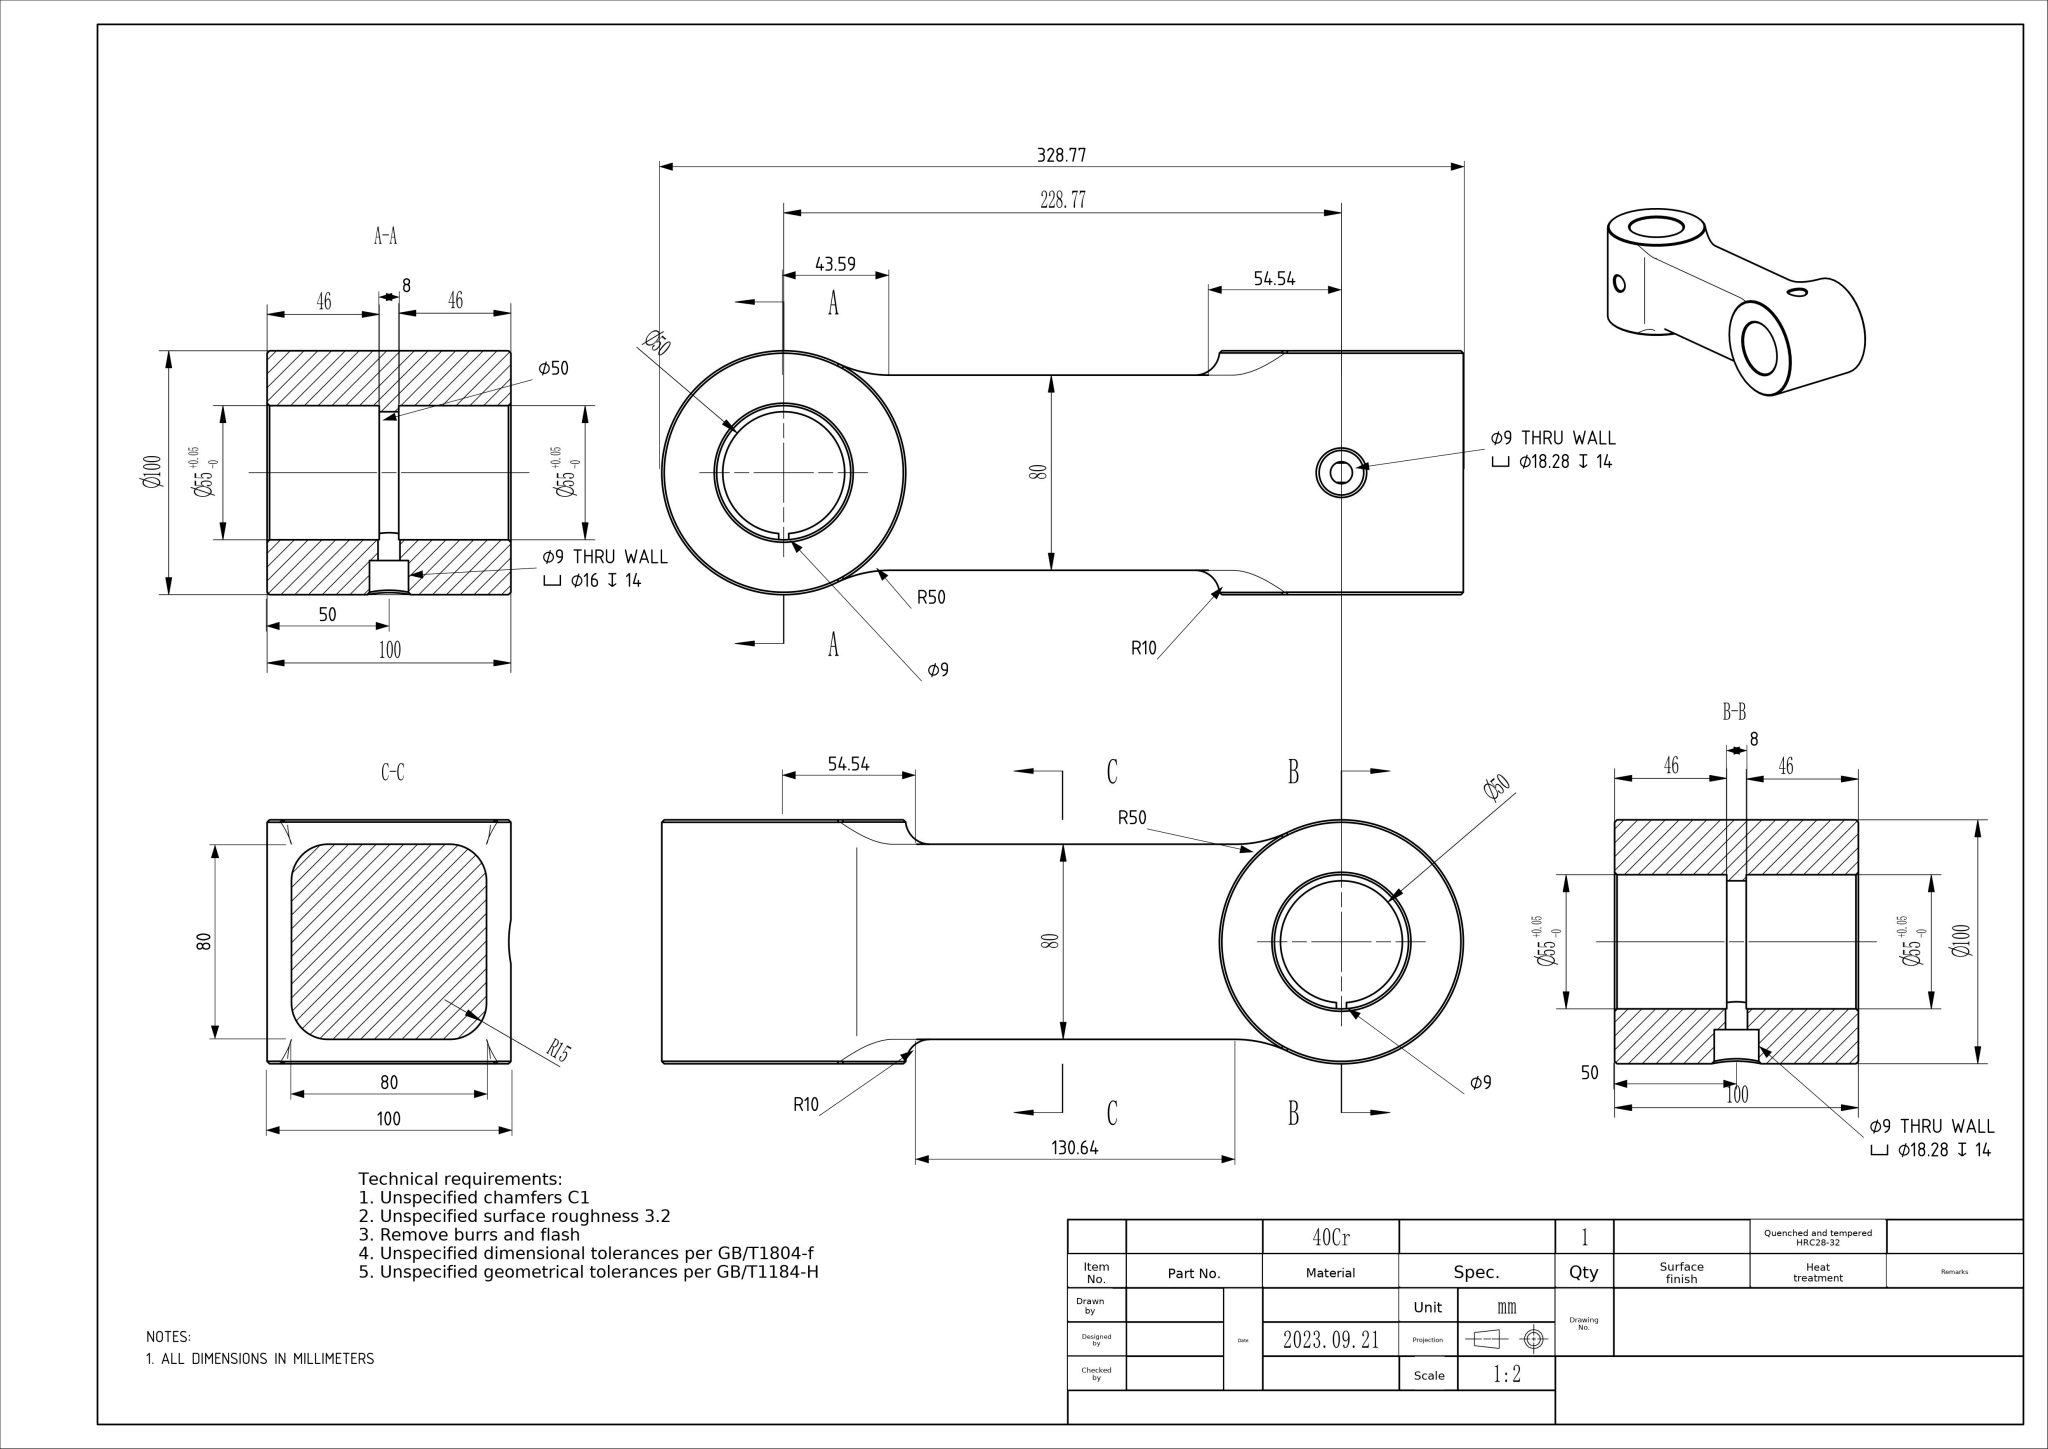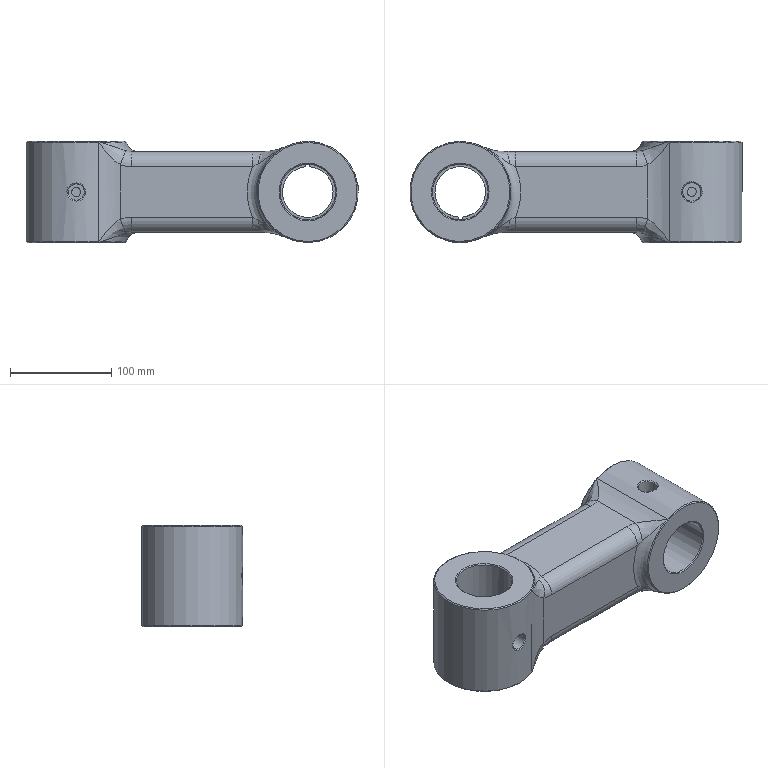Part | NX | mm | 1 solid | 84 faces | box 328.77 x 100 x 100 mm | volume 1979527 mm3 | spline 26 | cylinder 20 | cone 20 | plane 14 | torus 4 | commonest cylinder face diameters 100 x6 55 x4 30 x4 9 x2 50 x2 16 x1 18.281 x1